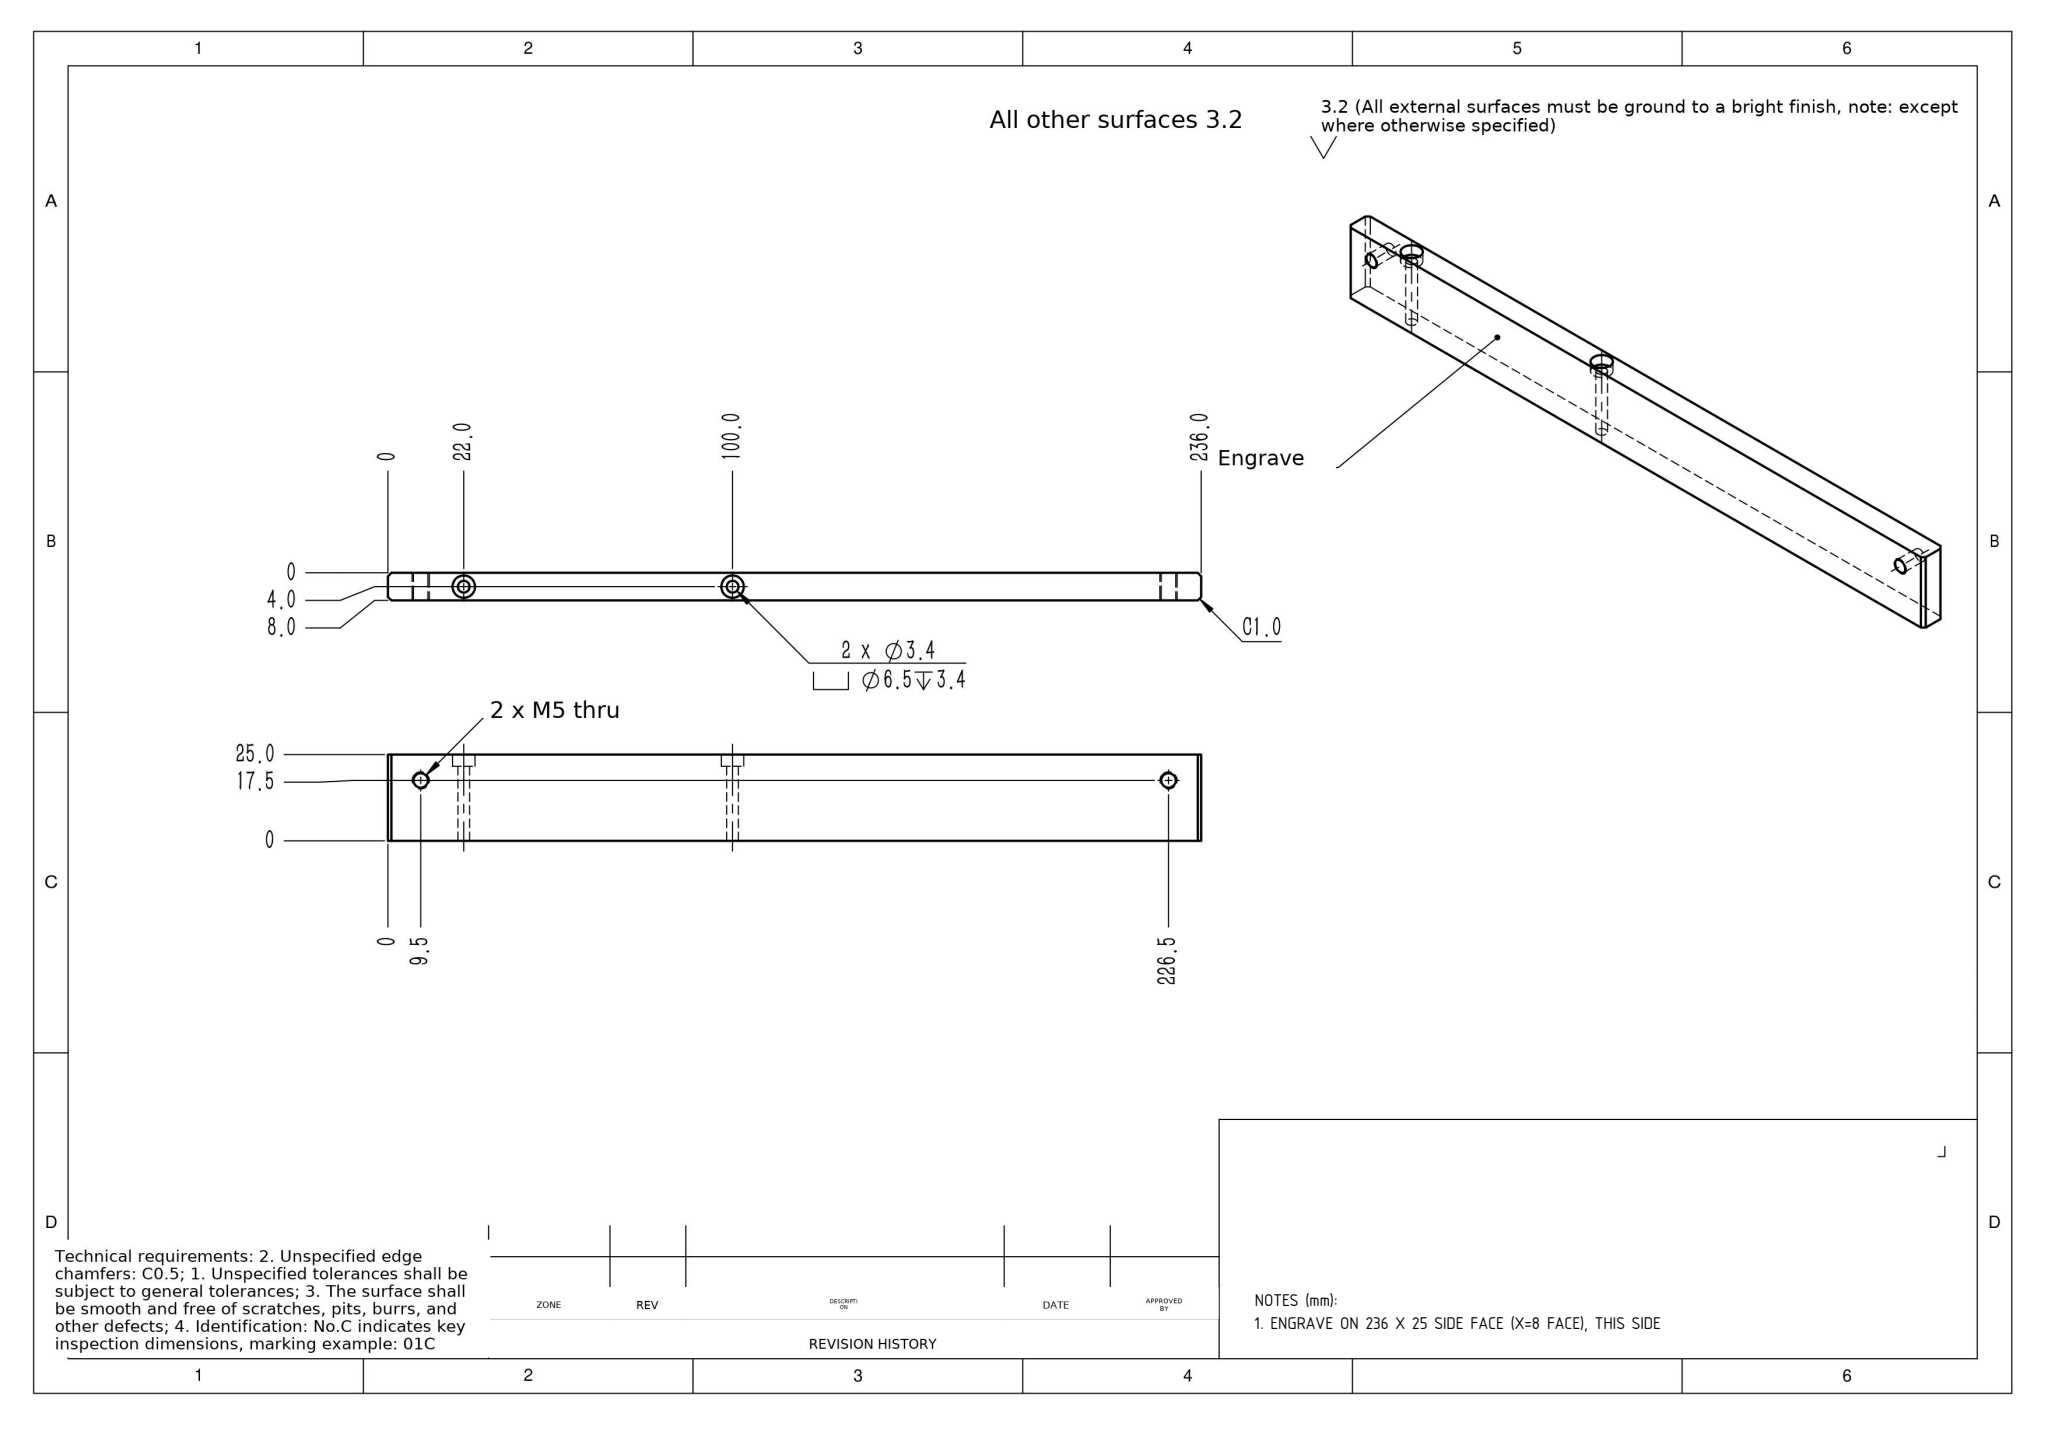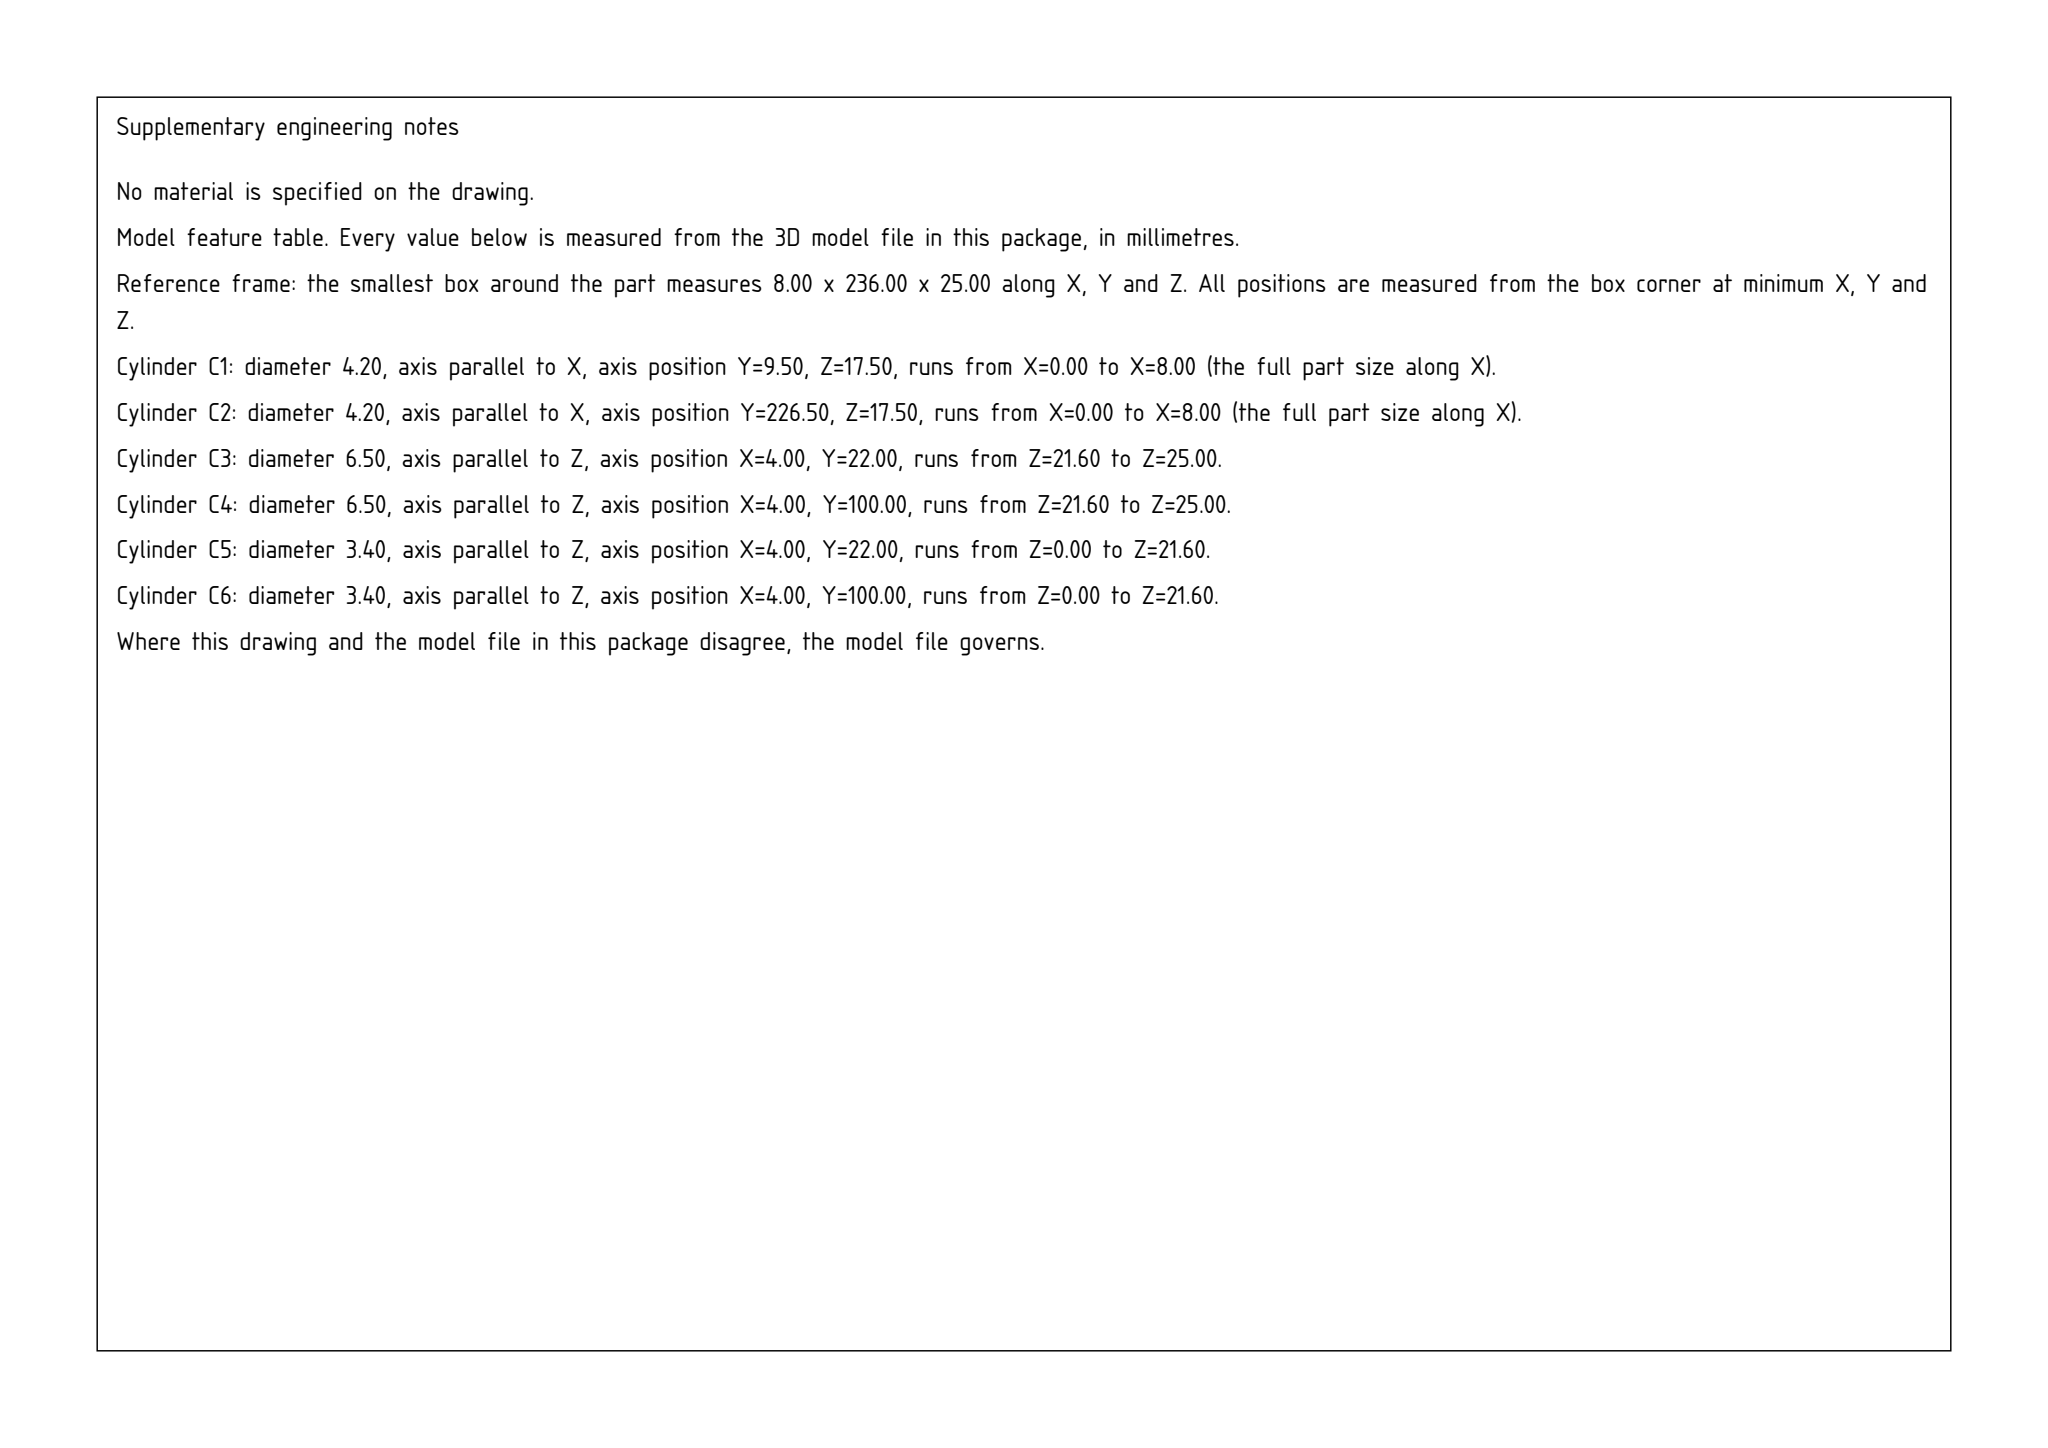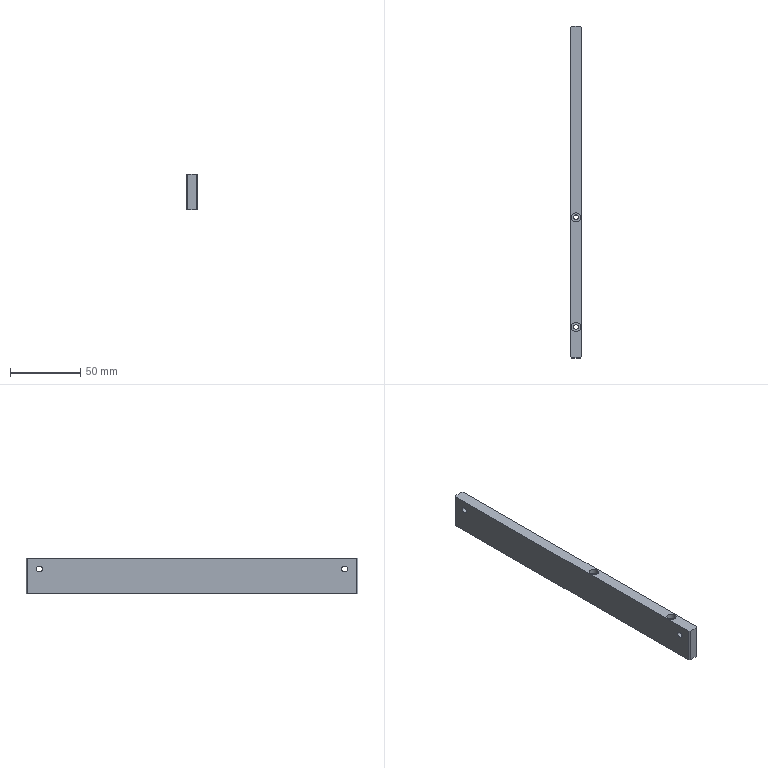Part | SolidWorks | mm | 1 solid | 24 faces | box 8 x 236 x 25 mm | volume 46310 mm3 | cylinder 12 | plane 12 | commonest cylinder face diameters 4.2 x4 6.5 x4 3.4 x4
Drawing notes:
ENGRAVE ON 236 X 25 SIDE FACE (X=8 FACE), THIS SIDE | from the solid: Planar face normal x at offset 8.0; bbox 8.0 x 236.0 x 25.0 gives 236x25 side face
build123d program:
from build123d import *

# Parameters (mm, degrees)
SKETCH1_W                                       = 8
SKETCH1_H                                       = 236
BOSS_EXTRUDE1_DEPTH                             = 25
M3_HEX_SOCKET_HEAD_CAP_SCREW_CBORE1_D           = 3.4
M3_HEX_SOCKET_HEAD_CAP_SCREW_CBORE1_CBORE_D     = 6.5
M3_HEX_SOCKET_HEAD_CAP_SCREW_CBORE1_CBORE_DEPTH = 3.4
M5_TAPPED_HOLE1_D                               = 4.2
CHAMFER1_SIZE                                   = 1


with BuildPart() as part:
    # Sketch1 → Boss-Extrude1 (new body)
    with BuildSketch(Plane.XY):
        Rectangle(SKETCH1_W, SKETCH1_H)
    extrude(amount=BOSS_EXTRUDE1_DEPTH)

    # M3 Hex Socket Head Cap Screw CBORE1 (through all)
    with Locations(Plane.XY.offset(25)):
        with Locations((0, -96), (0, -18)):
            CounterBoreHole(M3_HEX_SOCKET_HEAD_CAP_SCREW_CBORE1_D / 2, M3_HEX_SOCKET_HEAD_CAP_SCREW_CBORE1_CBORE_D / 2, M3_HEX_SOCKET_HEAD_CAP_SCREW_CBORE1_CBORE_DEPTH)

    # M5 Tapped Hole1 (through all)
    with Locations(Plane(origin=(4, 0, 0), x_dir=(0, 0, -1), z_dir=(1, 0, 0))):
        with Locations((-17.5, 108.5), (-17.5, -108.5)):
            Hole(M5_TAPPED_HOLE1_D / 2)

    # Chamfer1
    chamfer1_edges = [part.edges().sort_by_distance(p)[0] for p in [
        (4, -118, 12.5),
        (-4, -118, 12.5),
        (-4, 118, 12.5),
        (4, 118, 12.5),
    ]]
    chamfer(chamfer1_edges, length=CHAMFER1_SIZE)


solid = part.part
STEP:
#1=CARTESIAN_POINT('',(-4.,108.5,19.6));
#2=VERTEX_POINT('',#1);
#3=CARTESIAN_POINT('',(-4.,108.5,15.4));
#4=VERTEX_POINT('',#3);
#5=CARTESIAN_POINT('',(-4.,108.5,17.5));
#6=DIRECTION('',(1.,0.,0.));
#7=DIRECTION('',(0.,0.,-1.));
#8=AXIS2_PLACEMENT_3D('',#5,#6,#7);
#9=CIRCLE('',#8,2.1);
#10=EDGE_CURVE('',#2,#4,#9,.T.);
#11=ORIENTED_EDGE('',*,*,#10,.F.);
#12=CARTESIAN_POINT('',(4.,108.5,19.6));
#13=VERTEX_POINT('',#12);
#14=CARTESIAN_POINT('',(4.,108.5,19.6));
#15=DIRECTION('',(1.,0.,0.));
#16=VECTOR('',#15,1000.);
#17=LINE('',#14,#16);
#18=EDGE_CURVE('',#2,#13,#17,.T.);
#19=ORIENTED_EDGE('',*,*,#18,.T.);
#20=CARTESIAN_POINT('',(4.,108.5,15.4));
#21=VERTEX_POINT('',#20);
#22=CARTESIAN_POINT('',(4.,108.5,17.5));
#23=DIRECTION('',(1.,0.,0.));
#24=DIRECTION('',(0.,0.,-1.));
#25=AXIS2_PLACEMENT_3D('',#22,#23,#24);
#26=CIRCLE('',#25,2.1);
#27=EDGE_CURVE('',#13,#21,#26,.T.);
#28=ORIENTED_EDGE('',*,*,#27,.T.);
#29=CARTESIAN_POINT('',(4.,108.5,15.4));
#30=DIRECTION('',(1.,0.,0.));
#31=VECTOR('',#30,1000.);
#32=LINE('',#29,#31);
#33=EDGE_CURVE('',#4,#21,#32,.T.);
#34=ORIENTED_EDGE('',*,*,#33,.F.);
#35=EDGE_LOOP('',(#11,#19,#28,#34));
#36=FACE_OUTER_BOUND('',#35,.T.);
#37=CARTESIAN_POINT('',(4.,108.5,17.5));
#38=DIRECTION('',(1.,0.,0.));
#39=DIRECTION('',(0.,0.,-1.));
#40=AXIS2_PLACEMENT_3D('',#37,#38,#39);
#41=CYLINDRICAL_SURFACE('',#40,2.1);
#42=ADVANCED_FACE('',(#36),#41,.F.);
#43=CARTESIAN_POINT('',(-4.,-108.5,19.6));
#44=VERTEX_POINT('',#43);
#45=CARTESIAN_POINT('',(-4.,-108.5,15.4));
#46=VERTEX_POINT('',#45);
#47=CARTESIAN_POINT('',(-4.,-108.5,17.5));
#48=DIRECTION('',(1.,0.,0.));
#49=DIRECTION('',(0.,0.,-1.));
#50=AXIS2_PLACEMENT_3D('',#47,#48,#49);
#51=CIRCLE('',#50,2.1);
#52=EDGE_CURVE('',#44,#46,#51,.T.);
#53=ORIENTED_EDGE('',*,*,#52,.F.);
#54=CARTESIAN_POINT('',(4.,-108.5,19.6));
#55=VERTEX_POINT('',#54);
#56=CARTESIAN_POINT('',(4.,-108.5,19.6));
#57=DIRECTION('',(1.,0.,0.));
#58=VECTOR('',#57,1000.);
#59=LINE('',#56,#58);
#60=EDGE_CURVE('',#44,#55,#59,.T.);
#61=ORIENTED_EDGE('',*,*,#60,.T.);
#62=CARTESIAN_POINT('',(4.,-108.5,15.4));
#63=VERTEX_POINT('',#62);
#64=CARTESIAN_POINT('',(4.,-108.5,17.5));
#65=DIRECTION('',(1.,0.,0.));
#66=DIRECTION('',(0.,0.,-1.));
#67=AXIS2_PLACEMENT_3D('',#64,#65,#66);
#68=CIRCLE('',#67,2.1);
#69=EDGE_CURVE('',#55,#63,#68,.T.);
#70=ORIENTED_EDGE('',*,*,#69,.T.);
#71=CARTESIAN_POINT('',(4.,-108.5,15.4));
#72=DIRECTION('',(1.,0.,0.));
#73=VECTOR('',#72,1000.);
#74=LINE('',#71,#73);
#75=EDGE_CURVE('',#46,#63,#74,.T.);
#76=ORIENTED_EDGE('',*,*,#75,.F.);
#77=EDGE_LOOP('',(#53,#61,#70,#76));
#78=FACE_OUTER_BOUND('',#77,.T.);
#79=CARTESIAN_POINT('',(4.,-108.5,17.5));
#80=DIRECTION('',(1.,0.,0.));
#81=DIRECTION('',(0.,0.,-1.));
#82=AXIS2_PLACEMENT_3D('',#79,#80,#81);
#83=CYLINDRICAL_SURFACE('',#82,2.1);
#84=ADVANCED_FACE('',(#78),#83,.F.);
#85=CARTESIAN_POINT('',(-3.25,-96.,21.6));
#86=VERTEX_POINT('',#85);
#87=CARTESIAN_POINT('',(3.25,-96.,21.6));
#88=VERTEX_POINT('',#87);
#89=CARTESIAN_POINT('',(-0.,-96.,21.6));
#90=DIRECTION('',(0.,0.,1.));
#91=DIRECTION('',(1.,0.,0.));
#92=AXIS2_PLACEMENT_3D('',#89,#90,#91);
#93=CIRCLE('',#92,3.25);
#94=EDGE_CURVE('',#86,#88,#93,.T.);
#95=ORIENTED_EDGE('',*,*,#94,.F.);
#96=CARTESIAN_POINT('',(-3.25,-96.,25.));
#97=VERTEX_POINT('',#96);
#98=CARTESIAN_POINT('',(-3.25,-96.,25.));
#99=DIRECTION('',(0.,0.,1.));
#100=VECTOR('',#99,1000.);
#101=LINE('',#98,#100);
#102=EDGE_CURVE('',#86,#97,#101,.T.);
#103=ORIENTED_EDGE('',*,*,#102,.T.);
#104=CARTESIAN_POINT('',(3.25,-96.,25.));
#105=VERTEX_POINT('',#104);
#106=CARTESIAN_POINT('',(-0.,-96.,25.));
#107=DIRECTION('',(0.,0.,1.));
#108=DIRECTION('',(1.,0.,0.));
#109=AXIS2_PLACEMENT_3D('',#106,#107,#108);
#110=CIRCLE('',#109,3.25);
#111=EDGE_CURVE('',#97,#105,#110,.T.);
#112=ORIENTED_EDGE('',*,*,#111,.T.);
#113=CARTESIAN_POINT('',(3.25,-96.,25.));
#114=DIRECTION('',(0.,0.,1.));
#115=VECTOR('',#114,1000.);
#116=LINE('',#113,#115);
#117=EDGE_CURVE('',#88,#105,#116,.T.);
#118=ORIENTED_EDGE('',*,*,#117,.F.);
#119=EDGE_LOOP('',(#95,#103,#112,#118));
#120=FACE_OUTER_BOUND('',#119,.T.);
#121=CARTESIAN_POINT('',(-0.,-96.,25.));
#122=DIRECTION('',(0.,0.,1.));
#123=DIRECTION('',(1.,0.,0.));
#124=AXIS2_PLACEMENT_3D('',#121,#122,#123);
#125=CYLINDRICAL_SURFACE('',#124,3.25);
#126=ADVANCED_FACE('',(#120),#125,.F.);
#127=CARTESIAN_POINT('',(-1.7,-96.,0.));
#128=VERTEX_POINT('',#127);
#129=CARTESIAN_POINT('',(1.7,-96.,0.));
#130=VERTEX_POINT('',#129);
#131=CARTESIAN_POINT('',(-0.,-96.,0.));
#132=DIRECTION('',(0.,0.,1.));
#133=DIRECTION('',(1.,0.,0.));
#134=AXIS2_PLACEMENT_3D('',#131,#132,#133);
#135=CIRCLE('',#134,1.7);
#136=EDGE_CURVE('',#128,#130,#135,.T.);
#137=ORIENTED_EDGE('',*,*,#136,.F.);
#138=CARTESIAN_POINT('',(-1.7,-96.,21.6));
#139=VERTEX_POINT('',#138);
#140=CARTESIAN_POINT('',(-1.7,-96.,25.));
#141=DIRECTION('',(0.,0.,1.));
#142=VECTOR('',#141,1000.);
#143=LINE('',#140,#142);
#144=EDGE_CURVE('',#128,#139,#143,.T.);
#145=ORIENTED_EDGE('',*,*,#144,.T.);
#146=CARTESIAN_POINT('',(1.7,-96.,21.6));
#147=VERTEX_POINT('',#146);
#148=CARTESIAN_POINT('',(-0.,-96.,21.6));
#149=DIRECTION('',(0.,0.,1.));
#150=DIRECTION('',(1.,0.,0.));
#151=AXIS2_PLACEMENT_3D('',#148,#149,#150);
#152=CIRCLE('',#151,1.7);
#153=EDGE_CURVE('',#139,#147,#152,.T.);
#154=ORIENTED_EDGE('',*,*,#153,.T.);
#155=CARTESIAN_POINT('',(1.7,-96.,25.));
#156=DIRECTION('',(0.,0.,1.));
#157=VECTOR('',#156,1000.);
#158=LINE('',#155,#157);
#159=EDGE_CURVE('',#130,#147,#158,.T.);
#160=ORIENTED_EDGE('',*,*,#159,.F.);
#161=EDGE_LOOP('',(#137,#145,#154,#160));
#162=FACE_OUTER_BOUND('',#161,.T.);
#163=CARTESIAN_POINT('',(-0.,-96.,25.));
#164=DIRECTION('',(0.,0.,1.));
#165=DIRECTION('',(1.,0.,0.));
#166=AXIS2_PLACEMENT_3D('',#163,#164,#165);
#167=CYLINDRICAL_SURFACE('',#166,1.7);
#168=ADVANCED_FACE('',(#162),#167,.F.);
#169=CARTESIAN_POINT('',(-3.25,-18.,21.6));
#170=VERTEX_POINT('',#169);
#171=CARTESIAN_POINT('',(3.25,-18.,21.6));
#172=VERTEX_POINT('',#171);
#173=CARTESIAN_POINT('',(-0.,-18.,21.6));
#174=DIRECTION('',(0.,0.,1.));
#175=DIRECTION('',(1.,0.,0.));
#176=AXIS2_PLACEMENT_3D('',#173,#174,#175);
#177=CIRCLE('',#176,3.25);
#178=EDGE_CURVE('',#170,#172,#177,.T.);
#179=ORIENTED_EDGE('',*,*,#178,.F.);
#180=CARTESIAN_POINT('',(-3.25,-18.,25.));
#181=VERTEX_POINT('',#180);
#182=CARTESIAN_POINT('',(-3.25,-18.,25.));
#183=DIRECTION('',(0.,0.,1.));
#184=VECTOR('',#183,1000.);
#185=LINE('',#182,#184);
#186=EDGE_CURVE('',#170,#181,#185,.T.);
#187=ORIENTED_EDGE('',*,*,#186,.T.);
#188=CARTESIAN_POINT('',(3.25,-18.,25.));
#189=VERTEX_POINT('',#188);
#190=CARTESIAN_POINT('',(-0.,-18.,25.));
#191=DIRECTION('',(0.,0.,1.));
#192=DIRECTION('',(1.,0.,0.));
#193=AXIS2_PLACEMENT_3D('',#190,#191,#192);
#194=CIRCLE('',#193,3.25);
#195=EDGE_CURVE('',#181,#189,#194,.T.);
#196=ORIENTED_EDGE('',*,*,#195,.T.);
#197=CARTESIAN_POINT('',(3.25,-18.,25.));
#198=DIRECTION('',(0.,0.,1.));
#199=VECTOR('',#198,1000.);
#200=LINE('',#197,#199);
#201=EDGE_CURVE('',#172,#189,#200,.T.);
#202=ORIENTED_EDGE('',*,*,#201,.F.);
#203=EDGE_LOOP('',(#179,#187,#196,#202));
#204=FACE_OUTER_BOUND('',#203,.T.);
#205=CARTESIAN_POINT('',(-0.,-18.,25.));
#206=DIRECTION('',(0.,0.,1.));
#207=DIRECTION('',(1.,0.,0.));
#208=AXIS2_PLACEMENT_3D('',#205,#206,#207);
#209=CYLINDRICAL_SURFACE('',#208,3.25);
#210=ADVANCED_FACE('',(#204),#209,.F.);
#211=CARTESIAN_POINT('',(-1.7,-18.,0.));
#212=VERTEX_POINT('',#211);
#213=CARTESIAN_POINT('',(1.7,-18.,0.));
#214=VERTEX_POINT('',#213);
#215=CARTESIAN_POINT('',(-0.,-18.,0.));
#216=DIRECTION('',(0.,0.,1.));
#217=DIRECTION('',(1.,0.,0.));
#218=AXIS2_PLACEMENT_3D('',#215,#216,#217);
#219=CIRCLE('',#218,1.7);
#220=EDGE_CURVE('',#212,#214,#219,.T.);
#221=ORIENTED_EDGE('',*,*,#220,.F.);
#222=CARTESIAN_POINT('',(-1.7,-18.,21.6));
#223=VERTEX_POINT('',#222);
#224=CARTESIAN_POINT('',(-1.7,-18.,25.));
#225=DIRECTION('',(0.,0.,1.));
#226=VECTOR('',#225,1000.);
#227=LINE('',#224,#226);
#228=EDGE_CURVE('',#212,#223,#227,.T.);
#229=ORIENTED_EDGE('',*,*,#228,.T.);
#230=CARTESIAN_POINT('',(1.7,-18.,21.6));
#231=VERTEX_POINT('',#230);
#232=CARTESIAN_POINT('',(-0.,-18.,21.6));
#233=DIRECTION('',(0.,0.,1.));
#234=DIRECTION('',(1.,0.,0.));
#235=AXIS2_PLACEMENT_3D('',#232,#233,#234);
#236=CIRCLE('',#235,1.7);
#237=EDGE_CURVE('',#223,#231,#236,.T.);
#238=ORIENTED_EDGE('',*,*,#237,.T.);
#239=CARTESIAN_POINT('',(1.7,-18.,25.));
#240=DIRECTION('',(0.,0.,1.));
#241=VECTOR('',#240,1000.);
#242=LINE('',#239,#241);
#243=EDGE_CURVE('',#214,#231,#242,.T.);
#244=ORIENTED_EDGE('',*,*,#243,.F.);
#245=EDGE_LOOP('',(#221,#229,#238,#244));
#246=FACE_OUTER_BOUND('',#245,.T.);
#247=CARTESIAN_POINT('',(-0.,-18.,25.));
#248=DIRECTION('',(0.,0.,1.));
#249=DIRECTION('',(1.,0.,0.));
#250=AXIS2_PLACEMENT_3D('',#247,#248,#249);
#251=CYLINDRICAL_SURFACE('',#250,1.7);
#252=ADVANCED_FACE('',(#246),#251,.F.);
#253=CARTESIAN_POINT('',(4.,108.5,17.5));
#254=DIRECTION('',(1.,0.,0.));
#255=DIRECTION('',(0.,0.,-1.));
#256=AXIS2_PLACEMENT_3D('',#253,#254,#255);
#257=CIRCLE('',#256,2.1);
#258=EDGE_CURVE('',#21,#13,#257,.T.);
#259=ORIENTED_EDGE('',*,*,#258,.F.);
#260=ORIENTED_EDGE('',*,*,#27,.F.);
#261=EDGE_LOOP('',(#259,#260));
#262=FACE_BOUND('',#261,.T.);
#263=CARTESIAN_POINT('',(4.,-108.5,17.5));
#264=DIRECTION('',(1.,0.,0.));
#265=DIRECTION('',(0.,0.,-1.));
#266=AXIS2_PLACEMENT_3D('',#263,#264,#265);
#267=CIRCLE('',#266,2.1);
#268=EDGE_CURVE('',#63,#55,#267,.T.);
#269=ORIENTED_EDGE('',*,*,#268,.F.);
#270=ORIENTED_EDGE('',*,*,#69,.F.);
#271=EDGE_LOOP('',(#269,#270));
#272=FACE_BOUND('',#271,.T.);
#273=CARTESIAN_POINT('',(4.,-117.,25.));
#274=VERTEX_POINT('',#273);
#275=CARTESIAN_POINT('',(4.,117.,25.));
#276=VERTEX_POINT('',#275);
#277=CARTESIAN_POINT('',(4.,-118.,25.));
#278=DIRECTION('',(0.,1.,0.));
#279=VECTOR('',#278,1000.);
#280=LINE('',#277,#279);
#281=EDGE_CURVE('',#274,#276,#280,.T.);
#282=ORIENTED_EDGE('',*,*,#281,.F.);
#283=CARTESIAN_POINT('',(4.,-117.,0.));
#284=VERTEX_POINT('',#283);
#285=CARTESIAN_POINT('',(4.,-117.,25.));
#286=DIRECTION('',(0.,0.,-1.));
#287=VECTOR('',#286,1000.);
#288=LINE('',#285,#287);
#289=EDGE_CURVE('',#274,#284,#288,.T.);
#290=ORIENTED_EDGE('',*,*,#289,.T.);
#291=CARTESIAN_POINT('',(4.,117.,0.));
#292=VERTEX_POINT('',#291);
#293=CARTESIAN_POINT('',(4.,-118.,0.));
#294=DIRECTION('',(0.,1.,0.));
#295=VECTOR('',#294,1000.);
#296=LINE('',#293,#295);
#297=EDGE_CURVE('',#284,#292,#296,.T.);
#298=ORIENTED_EDGE('',*,*,#297,.T.);
#299=CARTESIAN_POINT('',(4.,117.,25.));
#300=DIRECTION('',(0.,0.,1.));
#301=VECTOR('',#300,1000.);
#302=LINE('',#299,#301);
#303=EDGE_CURVE('',#292,#276,#302,.T.);
#304=ORIENTED_EDGE('',*,*,#303,.T.);
#305=EDGE_LOOP('',(#282,#290,#298,#304));
#306=FACE_OUTER_BOUND('',#305,.T.);
#307=CARTESIAN_POINT('',(4.,-118.,25.));
#308=DIRECTION('',(-1.,0.,0.));
#309=DIRECTION('',(0.,0.,1.));
#310=AXIS2_PLACEMENT_3D('',#307,#308,#309);
#311=PLANE('',#310);
#312=ADVANCED_FACE('',(#262,#272,#306),#311,.F.);
#313=CARTESIAN_POINT('',(3.,118.,0.));
#314=VERTEX_POINT('',#313);
#315=CARTESIAN_POINT('',(-3.,118.,0.));
#316=VERTEX_POINT('',#315);
#317=CARTESIAN_POINT('',(-4.,118.,0.));
#318=DIRECTION('',(-1.,0.,0.));
#319=VECTOR('',#318,1000.);
#320=LINE('',#317,#319);
#321=EDGE_CURVE('',#314,#316,#320,.T.);
#322=ORIENTED_EDGE('',*,*,#321,.T.);
#323=CARTESIAN_POINT('',(-3.,118.,25.));
#324=VERTEX_POINT('',#323);
#325=CARTESIAN_POINT('',(-3.,118.,25.));
#326=DIRECTION('',(0.,0.,1.));
#327=VECTOR('',#326,1000.);
#328=LINE('',#325,#327);
#329=EDGE_CURVE('',#316,#324,#328,.T.);
#330=ORIENTED_EDGE('',*,*,#329,.T.);
#331=CARTESIAN_POINT('',(3.,118.,25.));
#332=VERTEX_POINT('',#331);
#333=CARTESIAN_POINT('',(-4.,118.,25.));
#334=DIRECTION('',(-1.,0.,0.));
#335=VECTOR('',#334,1000.);
#336=LINE('',#333,#335);
#337=EDGE_CURVE('',#332,#324,#336,.T.);
#338=ORIENTED_EDGE('',*,*,#337,.F.);
#339=CARTESIAN_POINT('',(3.,118.,25.));
#340=DIRECTION('',(0.,0.,-1.));
#341=VECTOR('',#340,1000.);
#342=LINE('',#339,#341);
#343=EDGE_CURVE('',#332,#314,#342,.T.);
#344=ORIENTED_EDGE('',*,*,#343,.T.);
#345=EDGE_LOOP('',(#322,#330,#338,#344));
#346=FACE_OUTER_BOUND('',#345,.T.);
#347=CARTESIAN_POINT('',(-4.,118.,25.));
#348=DIRECTION('',(0.,-1.,0.));
#349=DIRECTION('',(0.,0.,-1.));
#350=AXIS2_PLACEMENT_3D('',#347,#348,#349);
#351=PLANE('',#350);
#352=ADVANCED_FACE('',(#346),#351,.F.);
#353=CARTESIAN_POINT('',(-4.,108.5,17.5));
#354=DIRECTION('',(1.,0.,0.));
#355=DIRECTION('',(0.,0.,-1.));
#356=AXIS2_PLACEMENT_3D('',#353,#354,#355);
#357=CIRCLE('',#356,2.1);
#358=EDGE_CURVE('',#4,#2,#357,.T.);
#359=ORIENTED_EDGE('',*,*,#358,.T.);
#360=ORIENTED_EDGE('',*,*,#10,.T.);
#361=EDGE_LOOP('',(#359,#360));
#362=FACE_BOUND('',#361,.T.);
#363=CARTESIAN_POINT('',(-4.,-108.5,17.5));
#364=DIRECTION('',(1.,0.,0.));
#365=DIRECTION('',(0.,0.,-1.));
#366=AXIS2_PLACEMENT_3D('',#363,#364,#365);
#367=CIRCLE('',#366,2.1);
#368=EDGE_CURVE('',#46,#44,#367,.T.);
#369=ORIENTED_EDGE('',*,*,#368,.T.);
#370=ORIENTED_EDGE('',*,*,#52,.T.);
#371=EDGE_LOOP('',(#369,#370));
#372=FACE_BOUND('',#371,.T.);
#373=CARTESIAN_POINT('',(-4.,117.,0.));
#374=VERTEX_POINT('',#373);
#375=CARTESIAN_POINT('',(-4.,-117.,0.));
#376=VERTEX_POINT('',#375);
#377=CARTESIAN_POINT('',(-4.,-118.,0.));
#378=DIRECTION('',(0.,-1.,0.));
#379=VECTOR('',#378,1000.);
#380=LINE('',#377,#379);
#381=EDGE_CURVE('',#374,#376,#380,.T.);
#382=ORIENTED_EDGE('',*,*,#381,.T.);
#383=CARTESIAN_POINT('',(-4.,-117.,25.));
#384=VERTEX_POINT('',#383);
#385=CARTESIAN_POINT('',(-4.,-117.,25.));
#386=DIRECTION('',(0.,0.,1.));
#387=VECTOR('',#386,1000.);
#388=LINE('',#385,#387);
#389=EDGE_CURVE('',#376,#384,#388,.T.);
#390=ORIENTED_EDGE('',*,*,#389,.T.);
#391=CARTESIAN_POINT('',(-4.,117.,25.));
#392=VERTEX_POINT('',#391);
#393=CARTESIAN_POINT('',(-4.,-118.,25.));
#394=DIRECTION('',(0.,-1.,0.));
#395=VECTOR('',#394,1000.);
#396=LINE('',#393,#395);
#397=EDGE_CURVE('',#392,#384,#396,.T.);
#398=ORIENTED_EDGE('',*,*,#397,.F.);
#399=CARTESIAN_POINT('',(-4.,117.,25.));
#400=DIRECTION('',(0.,0.,-1.));
#401=VECTOR('',#400,1000.);
#402=LINE('',#399,#401);
#403=EDGE_CURVE('',#392,#374,#402,.T.);
#404=ORIENTED_EDGE('',*,*,#403,.T.);
#405=EDGE_LOOP('',(#382,#390,#398,#404));
#406=FACE_OUTER_BOUND('',#405,.T.);
#407=CARTESIAN_POINT('',(-4.,-118.,25.));
#408=DIRECTION('',(1.,0.,0.));
#409=DIRECTION('',(0.,0.,-1.));
#410=AXIS2_PLACEMENT_3D('',#407,#408,#409);
#411=PLANE('',#410);
#412=ADVANCED_FACE('',(#362,#372,#406),#411,.F.);
#413=CARTESIAN_POINT('',(-3.,-118.,25.));
#414=VERTEX_POINT('',#413);
#415=CARTESIAN_POINT('',(3.,-118.,25.));
#416=VERTEX_POINT('',#415);
#417=CARTESIAN_POINT('',(-4.,-118.,25.));
#418=DIRECTION('',(1.,0.,0.));
#419=VECTOR('',#418,1000.);
#420=LINE('',#417,#419);
#421=EDGE_CURVE('',#414,#416,#420,.T.);
#422=ORIENTED_EDGE('',*,*,#421,.F.);
#423=CARTESIAN_POINT('',(-3.,-118.,0.));
#424=VERTEX_POINT('',#423);
#425=CARTESIAN_POINT('',(-3.,-118.,25.));
#426=DIRECTION('',(0.,0.,-1.));
#427=VECTOR('',#426,1000.);
#428=LINE('',#425,#427);
#429=EDGE_CURVE('',#414,#424,#428,.T.);
#430=ORIENTED_EDGE('',*,*,#429,.T.);
#431=CARTESIAN_POINT('',(3.,-118.,0.));
#432=VERTEX_POINT('',#431);
#433=CARTESIAN_POINT('',(-4.,-118.,0.));
#434=DIRECTION('',(1.,0.,0.));
#435=VECTOR('',#434,1000.);
#436=LINE('',#433,#435);
#437=EDGE_CURVE('',#424,#432,#436,.T.);
#438=ORIENTED_EDGE('',*,*,#437,.T.);
#439=CARTESIAN_POINT('',(3.,-118.,25.));
#440=DIRECTION('',(0.,0.,1.));
#441=VECTOR('',#440,1000.);
#442=LINE('',#439,#441);
#443=EDGE_CURVE('',#432,#416,#442,.T.);
#444=ORIENTED_EDGE('',*,*,#443,.T.);
#445=EDGE_LOOP('',(#422,#430,#438,#444));
#446=FACE_OUTER_BOUND('',#445,.T.);
#447=CARTESIAN_POINT('',(-4.,-118.,25.));
#448=DIRECTION('',(0.,1.,0.));
#449=DIRECTION('',(0.,0.,1.));
#450=AXIS2_PLACEMENT_3D('',#447,#448,#449);
#451=PLANE('',#450);
#452=ADVANCED_FACE('',(#446),#451,.F.);
#453=CARTESIAN_POINT('',(-0.,-96.,25.));
#454=DIRECTION('',(0.,0.,1.));
#455=DIRECTION('',(1.,0.,0.));
#456=AXIS2_PLACEMENT_3D('',#453,#454,#455);
#457=CIRCLE('',#456,3.25);
#458=EDGE_CURVE('',#105,#97,#457,.T.);
#459=ORIENTED_EDGE('',*,*,#458,.F.);
#460=ORIENTED_EDGE('',*,*,#111,.F.);
#461=EDGE_LOOP('',(#459,#460));
#462=FACE_BOUND('',#461,.T.);
#463=CARTESIAN_POINT('',(-0.,-18.,25.));
#464=DIRECTION('',(0.,0.,1.));
#465=DIRECTION('',(1.,0.,0.));
#466=AXIS2_PLACEMENT_3D('',#463,#464,#465);
#467=CIRCLE('',#466,3.25);
#468=EDGE_CURVE('',#189,#181,#467,.T.);
#469=ORIENTED_EDGE('',*,*,#468,.F.);
#470=ORIENTED_EDGE('',*,*,#195,.F.);
#471=EDGE_LOOP('',(#469,#470));
#472=FACE_BOUND('',#471,.T.);
#473=ORIENTED_EDGE('',*,*,#397,.T.);
#474=CARTESIAN_POINT('',(-3.,-118.,25.));
#475=DIRECTION('',(0.7071,-0.7071,0.));
#476=VECTOR('',#475,1000.);
#477=LINE('',#474,#476);
#478=EDGE_CURVE('',#384,#414,#477,.T.);
#479=ORIENTED_EDGE('',*,*,#478,.T.);
#480=ORIENTED_EDGE('',*,*,#421,.T.);
#481=CARTESIAN_POINT('',(4.,-117.,25.));
#482=DIRECTION('',(0.7071,0.7071,0.));
#483=VECTOR('',#482,1000.);
#484=LINE('',#481,#483);
#485=EDGE_CURVE('',#416,#274,#484,.T.);
#486=ORIENTED_EDGE('',*,*,#485,.T.);
#487=ORIENTED_EDGE('',*,*,#281,.T.);
#488=CARTESIAN_POINT('',(3.,118.,25.));
#489=DIRECTION('',(-0.7071,0.7071,0.));
#490=VECTOR('',#489,1000.);
#491=LINE('',#488,#490);
#492=EDGE_CURVE('',#276,#332,#491,.T.);
#493=ORIENTED_EDGE('',*,*,#492,.T.);
#494=ORIENTED_EDGE('',*,*,#337,.T.);
#495=CARTESIAN_POINT('',(-4.,117.,25.));
#496=DIRECTION('',(-0.7071,-0.7071,0.));
#497=VECTOR('',#496,1000.);
#498=LINE('',#495,#497);
#499=EDGE_CURVE('',#324,#392,#498,.T.);
#500=ORIENTED_EDGE('',*,*,#499,.T.);
#501=EDGE_LOOP('',(#473,#479,#480,#486,#487,#493,#494,#500));
#502=FACE_OUTER_BOUND('',#501,.T.);
#503=CARTESIAN_POINT('',(0.,0.,25.));
#504=DIRECTION('',(0.,0.,-1.));
#505=DIRECTION('',(-1.,0.,0.));
#506=AXIS2_PLACEMENT_3D('',#503,#504,#505);
#507=PLANE('',#506);
#508=ADVANCED_FACE('',(#462,#472,#502),#507,.F.);
#509=CARTESIAN_POINT('',(-0.,-96.,0.));
#510=DIRECTION('',(0.,0.,1.));
#511=DIRECTION('',(1.,0.,0.));
#512=AXIS2_PLACEMENT_3D('',#509,#510,#511);
#513=CIRCLE('',#512,1.7);
#514=EDGE_CURVE('',#130,#128,#513,.T.);
#515=ORIENTED_EDGE('',*,*,#514,.T.);
#516=ORIENTED_EDGE('',*,*,#136,.T.);
#517=EDGE_LOOP('',(#515,#516));
#518=FACE_BOUND('',#517,.T.);
#519=CARTESIAN_POINT('',(-0.,-18.,0.));
#520=DIRECTION('',(0.,0.,1.));
#521=DIRECTION('',(1.,0.,0.));
#522=AXIS2_PLACEMENT_3D('',#519,#520,#521);
#523=CIRCLE('',#522,1.7);
#524=EDGE_CURVE('',#214,#212,#523,.T.);
#525=ORIENTED_EDGE('',*,*,#524,.T.);
#526=ORIENTED_EDGE('',*,*,#220,.T.);
#527=EDGE_LOOP('',(#525,#526));
#528=FACE_BOUND('',#527,.T.);
#529=ORIENTED_EDGE('',*,*,#437,.F.);
#530=CARTESIAN_POINT('',(-60.5,-60.5,0.));
#531=DIRECTION('',(-0.7071,0.7071,0.));
#532=VECTOR('',#531,1000.);
#533=LINE('',#530,#532);
#534=EDGE_CURVE('',#424,#376,#533,.T.);
#535=ORIENTED_EDGE('',*,*,#534,.T.);
#536=ORIENTED_EDGE('',*,*,#381,.F.);
#537=CARTESIAN_POINT('',(-60.5,60.5,0.));
#538=DIRECTION('',(0.7071,0.7071,0.));
#539=VECTOR('',#538,1000.);
#540=LINE('',#537,#539);
#541=EDGE_CURVE('',#374,#316,#540,.T.);
#542=ORIENTED_EDGE('',*,*,#541,.T.);
#543=ORIENTED_EDGE('',*,*,#321,.F.);
#544=CARTESIAN_POINT('',(60.5,60.5,0.));
#545=DIRECTION('',(0.7071,-0.7071,0.));
#546=VECTOR('',#545,1000.);
#547=LINE('',#544,#546);
#548=EDGE_CURVE('',#314,#292,#547,.T.);
#549=ORIENTED_EDGE('',*,*,#548,.T.);
#550=ORIENTED_EDGE('',*,*,#297,.F.);
#551=CARTESIAN_POINT('',(60.5,-60.5,0.));
#552=DIRECTION('',(-0.7071,-0.7071,0.));
#553=VECTOR('',#552,1000.);
#554=LINE('',#551,#553);
#555=EDGE_CURVE('',#284,#432,#554,.T.);
#556=ORIENTED_EDGE('',*,*,#555,.T.);
#557=EDGE_LOOP('',(#529,#535,#536,#542,#543,#549,#550,#556));
#558=FACE_OUTER_BOUND('',#557,.T.);
#559=CARTESIAN_POINT('',(0.,0.,0.));
#560=DIRECTION('',(0.,0.,-1.));
#561=DIRECTION('',(-1.,0.,0.));
#562=AXIS2_PLACEMENT_3D('',#559,#560,#561);
#563=PLANE('',#562);
#564=ADVANCED_FACE('',(#518,#528,#558),#563,.T.);
#565=ORIENTED_EDGE('',*,*,#228,.F.);
#566=ORIENTED_EDGE('',*,*,#524,.F.);
#567=ORIENTED_EDGE('',*,*,#243,.T.);
#568=CARTESIAN_POINT('',(-0.,-18.,21.6));
#569=DIRECTION('',(0.,0.,1.));
#570=DIRECTION('',(1.,0.,0.));
#571=AXIS2_PLACEMENT_3D('',#568,#569,#570);
#572=CIRCLE('',#571,1.7);
#573=EDGE_CURVE('',#231,#223,#572,.T.);
#574=ORIENTED_EDGE('',*,*,#573,.T.);
#575=EDGE_LOOP('',(#565,#566,#567,#574));
#576=FACE_OUTER_BOUND('',#575,.T.);
#577=CARTESIAN_POINT('',(-0.,-18.,25.));
#578=DIRECTION('',(0.,0.,1.));
#579=DIRECTION('',(1.,0.,0.));
#580=AXIS2_PLACEMENT_3D('',#577,#578,#579);
#581=CYLINDRICAL_SURFACE('',#580,1.7);
#582=ADVANCED_FACE('',(#576),#581,.F.);
#583=ORIENTED_EDGE('',*,*,#573,.F.);
#584=ORIENTED_EDGE('',*,*,#237,.F.);
#585=EDGE_LOOP('',(#583,#584));
#586=FACE_BOUND('',#585,.T.);
#587=CARTESIAN_POINT('',(-0.,-18.,21.6));
#588=DIRECTION('',(0.,0.,1.));
#589=DIRECTION('',(1.,0.,0.));
#590=AXIS2_PLACEMENT_3D('',#587,#588,#589);
#591=CIRCLE('',#590,3.25);
#592=EDGE_CURVE('',#172,#170,#591,.T.);
#593=ORIENTED_EDGE('',*,*,#592,.T.);
#594=ORIENTED_EDGE('',*,*,#178,.T.);
#595=EDGE_LOOP('',(#593,#594));
#596=FACE_OUTER_BOUND('',#595,.T.);
#597=CARTESIAN_POINT('',(1.7,-18.,21.6));
#598=DIRECTION('',(0.,0.,-1.));
#599=DIRECTION('',(-1.,0.,0.));
#600=AXIS2_PLACEMENT_3D('',#597,#598,#599);
#601=PLANE('',#600);
#602=ADVANCED_FACE('',(#586,#596),#601,.F.);
#603=ORIENTED_EDGE('',*,*,#186,.F.);
#604=ORIENTED_EDGE('',*,*,#592,.F.);
#605=ORIENTED_EDGE('',*,*,#201,.T.);
#606=ORIENTED_EDGE('',*,*,#468,.T.);
#607=EDGE_LOOP('',(#603,#604,#605,#606));
#608=FACE_OUTER_BOUND('',#607,.T.);
#609=CARTESIAN_POINT('',(-0.,-18.,25.));
#610=DIRECTION('',(0.,0.,1.));
#611=DIRECTION('',(1.,0.,0.));
#612=AXIS2_PLACEMENT_3D('',#609,#610,#611);
#613=CYLINDRICAL_SURFACE('',#612,3.25);
#614=ADVANCED_FACE('',(#608),#613,.F.);
#615=ORIENTED_EDGE('',*,*,#144,.F.);
#616=ORIENTED_EDGE('',*,*,#514,.F.);
#617=ORIENTED_EDGE('',*,*,#159,.T.);
#618=CARTESIAN_POINT('',(-0.,-96.,21.6));
#619=DIRECTION('',(0.,0.,1.));
#620=DIRECTION('',(1.,0.,0.));
#621=AXIS2_PLACEMENT_3D('',#618,#619,#620);
#622=CIRCLE('',#621,1.7);
#623=EDGE_CURVE('',#147,#139,#622,.T.);
#624=ORIENTED_EDGE('',*,*,#623,.T.);
#625=EDGE_LOOP('',(#615,#616,#617,#624));
#626=FACE_OUTER_BOUND('',#625,.T.);
#627=CARTESIAN_POINT('',(-0.,-96.,25.));
#628=DIRECTION('',(0.,0.,1.));
#629=DIRECTION('',(1.,0.,0.));
#630=AXIS2_PLACEMENT_3D('',#627,#628,#629);
#631=CYLINDRICAL_SURFACE('',#630,1.7);
#632=ADVANCED_FACE('',(#626),#631,.F.);
#633=ORIENTED_EDGE('',*,*,#623,.F.);
#634=ORIENTED_EDGE('',*,*,#153,.F.);
#635=EDGE_LOOP('',(#633,#634));
#636=FACE_BOUND('',#635,.T.);
#637=CARTESIAN_POINT('',(-0.,-96.,21.6));
#638=DIRECTION('',(0.,0.,1.));
#639=DIRECTION('',(1.,0.,0.));
#640=AXIS2_PLACEMENT_3D('',#637,#638,#639);
#641=CIRCLE('',#640,3.25);
#642=EDGE_CURVE('',#88,#86,#641,.T.);
#643=ORIENTED_EDGE('',*,*,#642,.T.);
#644=ORIENTED_EDGE('',*,*,#94,.T.);
#645=EDGE_LOOP('',(#643,#644));
#646=FACE_OUTER_BOUND('',#645,.T.);
#647=CARTESIAN_POINT('',(1.7,-96.,21.6));
#648=DIRECTION('',(0.,0.,-1.));
#649=DIRECTION('',(-1.,0.,0.));
#650=AXIS2_PLACEMENT_3D('',#647,#648,#649);
#651=PLANE('',#650);
#652=ADVANCED_FACE('',(#636,#646),#651,.F.);
#653=ORIENTED_EDGE('',*,*,#102,.F.);
#654=ORIENTED_EDGE('',*,*,#642,.F.);
#655=ORIENTED_EDGE('',*,*,#117,.T.);
#656=ORIENTED_EDGE('',*,*,#458,.T.);
#657=EDGE_LOOP('',(#653,#654,#655,#656));
#658=FACE_OUTER_BOUND('',#657,.T.);
#659=CARTESIAN_POINT('',(-0.,-96.,25.));
#660=DIRECTION('',(0.,0.,1.));
#661=DIRECTION('',(1.,0.,0.));
#662=AXIS2_PLACEMENT_3D('',#659,#660,#661);
#663=CYLINDRICAL_SURFACE('',#662,3.25);
#664=ADVANCED_FACE('',(#658),#663,.F.);
#665=ORIENTED_EDGE('',*,*,#60,.F.);
#666=ORIENTED_EDGE('',*,*,#368,.F.);
#667=ORIENTED_EDGE('',*,*,#75,.T.);
#668=ORIENTED_EDGE('',*,*,#268,.T.);
#669=EDGE_LOOP('',(#665,#666,#667,#668));
#670=FACE_OUTER_BOUND('',#669,.T.);
#671=CARTESIAN_POINT('',(4.,-108.5,17.5));
#672=DIRECTION('',(1.,0.,0.));
#673=DIRECTION('',(0.,0.,-1.));
#674=AXIS2_PLACEMENT_3D('',#671,#672,#673);
#675=CYLINDRICAL_SURFACE('',#674,2.1);
#676=ADVANCED_FACE('',(#670),#675,.F.);
#677=ORIENTED_EDGE('',*,*,#18,.F.);
#678=ORIENTED_EDGE('',*,*,#358,.F.);
#679=ORIENTED_EDGE('',*,*,#33,.T.);
#680=ORIENTED_EDGE('',*,*,#258,.T.);
#681=EDGE_LOOP('',(#677,#678,#679,#680));
#682=FACE_OUTER_BOUND('',#681,.T.);
#683=CARTESIAN_POINT('',(4.,108.5,17.5));
#684=DIRECTION('',(1.,0.,0.));
#685=DIRECTION('',(0.,0.,-1.));
#686=AXIS2_PLACEMENT_3D('',#683,#684,#685);
#687=CYLINDRICAL_SURFACE('',#686,2.1);
#688=ADVANCED_FACE('',(#682),#687,.F.);
#689=ORIENTED_EDGE('',*,*,#478,.F.);
#690=ORIENTED_EDGE('',*,*,#389,.F.);
#691=ORIENTED_EDGE('',*,*,#534,.F.);
#692=ORIENTED_EDGE('',*,*,#429,.F.);
#693=EDGE_LOOP('',(#689,#690,#691,#692));
#694=FACE_OUTER_BOUND('',#693,.T.);
#695=CARTESIAN_POINT('',(-3.,-118.,25.));
#696=DIRECTION('',(0.7071,0.7071,0.));
#697=DIRECTION('',(0.,0.,-1.));
#698=AXIS2_PLACEMENT_3D('',#695,#696,#697);
#699=PLANE('',#698);
#700=ADVANCED_FACE('',(#694),#699,.F.);
#701=ORIENTED_EDGE('',*,*,#485,.F.);
#702=ORIENTED_EDGE('',*,*,#443,.F.);
#703=ORIENTED_EDGE('',*,*,#555,.F.);
#704=ORIENTED_EDGE('',*,*,#289,.F.);
#705=EDGE_LOOP('',(#701,#702,#703,#704));
#706=FACE_OUTER_BOUND('',#705,.T.);
#707=CARTESIAN_POINT('',(4.,-117.,25.));
#708=DIRECTION('',(-0.7071,0.7071,0.));
#709=DIRECTION('',(0.,0.,-1.));
#710=AXIS2_PLACEMENT_3D('',#707,#708,#709);
#711=PLANE('',#710);
#712=ADVANCED_FACE('',(#706),#711,.F.);
#713=ORIENTED_EDGE('',*,*,#499,.F.);
#714=ORIENTED_EDGE('',*,*,#329,.F.);
#715=ORIENTED_EDGE('',*,*,#541,.F.);
#716=ORIENTED_EDGE('',*,*,#403,.F.);
#717=EDGE_LOOP('',(#713,#714,#715,#716));
#718=FACE_OUTER_BOUND('',#717,.T.);
#719=CARTESIAN_POINT('',(-4.,117.,25.));
#720=DIRECTION('',(0.7071,-0.7071,0.));
#721=DIRECTION('',(0.,0.,-1.));
#722=AXIS2_PLACEMENT_3D('',#719,#720,#721);
#723=PLANE('',#722);
#724=ADVANCED_FACE('',(#718),#723,.F.);
#725=ORIENTED_EDGE('',*,*,#492,.F.);
#726=ORIENTED_EDGE('',*,*,#303,.F.);
#727=ORIENTED_EDGE('',*,*,#548,.F.);
#728=ORIENTED_EDGE('',*,*,#343,.F.);
#729=EDGE_LOOP('',(#725,#726,#727,#728));
#730=FACE_OUTER_BOUND('',#729,.T.);
#731=CARTESIAN_POINT('',(3.,118.,25.));
#732=DIRECTION('',(-0.7071,-0.7071,0.));
#733=DIRECTION('',(0.,0.,-1.));
#734=AXIS2_PLACEMENT_3D('',#731,#732,#733);
#735=PLANE('',#734);
#736=ADVANCED_FACE('',(#730),#735,.F.);
#737=CLOSED_SHELL('',(#42,#84,#126,#168,#210,#252,#312,#352,#412,#452,#508,#564,#582,#602,#614,#632,#652,#664,#676,#688,#700,#712,#724,#736));
#738=MANIFOLD_SOLID_BREP('',#737);
#739=CARTESIAN_POINT('',(0.,0.,0.));
#740=DIRECTION('',(0.,0.,1.));
#741=DIRECTION('',(1.,0.,0.));
#742=AXIS2_PLACEMENT_3D('',#739,#740,#741);
#743=(LENGTH_UNIT()NAMED_UNIT(*)SI_UNIT(.MILLI.,.METRE.));
#744=UNCERTAINTY_MEASURE_WITH_UNIT(LENGTH_MEASURE(0.00001),#743,'','');
#745=(NAMED_UNIT(*)PLANE_ANGLE_UNIT()SI_UNIT($,.RADIAN.));
#746=(NAMED_UNIT(*)SI_UNIT($,.STERADIAN.)SOLID_ANGLE_UNIT());
#747=(GEOMETRIC_REPRESENTATION_CONTEXT(3)GLOBAL_UNCERTAINTY_ASSIGNED_CONTEXT((#744))GLOBAL_UNIT_ASSIGNED_CONTEXT((#743,#745,#746))REPRESENTATION_CONTEXT('',''));
#748=ADVANCED_BREP_SHAPE_REPRESENTATION('',(#738,#742),#747);